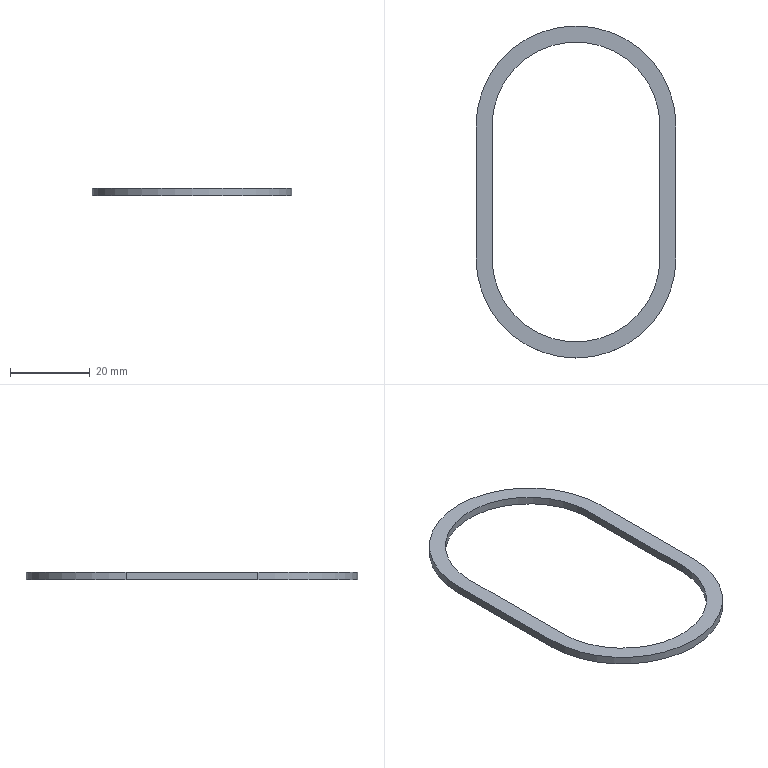Component | NX | 13 | 1 solid | 10 faces | box 50 x 83 x 2 mm | volume 1684 mm3 | plane 6 | cylinder 4 | commonest cylinder face diameters 42 x2 50 x2
STEP:
#1=CARTESIAN_POINT('',(0.,0.,0.));
#2=DIRECTION('',(0.,0.,1.));
#3=DIRECTION('',(1.,0.,0.));
#4=AXIS2_PLACEMENT_3D('',#1,#2,#3);
#5=CARTESIAN_POINT('',(-21.,16.5,30.));
#6=VERTEX_POINT('',#5);
#7=CARTESIAN_POINT('',(-21.,16.5,28.));
#8=VERTEX_POINT('',#7);
#9=CARTESIAN_POINT('',(-21.,16.5,30.));
#10=DIRECTION('',(0.,0.,-1.));
#11=VECTOR('',#10,1.);
#12=LINE('',#9,#11);
#13=CARTESIAN_POINT('',(0.0000016,16.5,30.));
#14=DIRECTION('',(0.,0.,-1.));
#15=DIRECTION('',(0.00000005,1.,0.));
#16=AXIS2_PLACEMENT_3D('',#13,#14,#15);
#17=CYLINDRICAL_SURFACE('',#16,21.);
#18=CARTESIAN_POINT('',(4.712,0.));
#19=DIRECTION('',(0.,1.));
#20=VECTOR('',#19,1.);
#21=LINE('',#18,#20);
#22=(GEOMETRIC_REPRESENTATION_CONTEXT(2)PARAMETRIC_REPRESENTATION_CONTEXT()REPRESENTATION_CONTEXT('',''));
#23=DEFINITIONAL_REPRESENTATION('',(#21),#22);
#24=PCURVE('',#17,#23);
#25=CARTESIAN_POINT('',(-21.,-16.5,30.));
#26=DIRECTION('',(-1.,0.00000005,0.));
#27=DIRECTION('',(-0.00000005,-1.,0.));
#28=AXIS2_PLACEMENT_3D('',#25,#26,#27);
#29=PLANE('',#28);
#30=CARTESIAN_POINT('',(-33.,0.));
#31=DIRECTION('',(0.,-1.));
#32=VECTOR('',#31,1.);
#33=LINE('',#30,#32);
#34=(GEOMETRIC_REPRESENTATION_CONTEXT(2)PARAMETRIC_REPRESENTATION_CONTEXT()REPRESENTATION_CONTEXT('',''));
#35=DEFINITIONAL_REPRESENTATION('',(#33),#34);
#36=PCURVE('',#29,#35);
#37=SURFACE_CURVE('',#12,(#24,#36),.PCURVE_S1.);
#38=EDGE_CURVE('',#6,#8,#37,.T.);
#39=ORIENTED_EDGE('',*,*,#38,.F.);
#40=CARTESIAN_POINT('',(21.,16.5,30.));
#41=VERTEX_POINT('',#40);
#42=CARTESIAN_POINT('',(0.0000016,16.5,30.));
#43=DIRECTION('',(0.,0.,-1.));
#44=DIRECTION('',(-0.00000005,-1.,0.));
#45=AXIS2_PLACEMENT_3D('',#42,#43,#44);
#46=CIRCLE('',#45,21.);
#47=CARTESIAN_POINT('',(3.142,0.));
#48=DIRECTION('',(1.,0.));
#49=VECTOR('',#48,1.);
#50=LINE('',#47,#49);
#51=(GEOMETRIC_REPRESENTATION_CONTEXT(2)PARAMETRIC_REPRESENTATION_CONTEXT()REPRESENTATION_CONTEXT('',''));
#52=DEFINITIONAL_REPRESENTATION('',(#50),#51);
#53=PCURVE('',#17,#52);
#54=CARTESIAN_POINT('',(0.0000016,16.5,30.));
#55=DIRECTION('',(0.,0.,1.));
#56=DIRECTION('',(-0.00000005,-1.,0.));
#57=AXIS2_PLACEMENT_3D('',#54,#55,#56);
#58=PLANE('',#57);
#59=CARTESIAN_POINT('',(21.,0.));
#60=CARTESIAN_POINT('',(21.,-36.373));
#61=CARTESIAN_POINT('',(-10.5,-18.187));
#62=CARTESIAN_POINT('',(-42.,-0.));
#63=CARTESIAN_POINT('',(-10.5,18.187));
#64=CARTESIAN_POINT('',(21.,36.373));
#65=CARTESIAN_POINT('',(21.,0.));
#66=(BOUNDED_CURVE()B_SPLINE_CURVE(2,(#59,#60,#61,#62,#63,#64,#65),.UNSPECIFIED.,.T.,.F.)B_SPLINE_CURVE_WITH_KNOTS((1,2,2,2,2,1),(-2.094,0.,2.094,4.189,6.283,8.378),.UNSPECIFIED.)CURVE()GEOMETRIC_REPRESENTATION_ITEM()RATIONAL_B_SPLINE_CURVE((1.,0.5,1.,0.5,1.,0.5,1.))REPRESENTATION_ITEM(''));
#67=(GEOMETRIC_REPRESENTATION_CONTEXT(2)PARAMETRIC_REPRESENTATION_CONTEXT()REPRESENTATION_CONTEXT('',''));
#68=DEFINITIONAL_REPRESENTATION('',(#66),#67);
#69=PCURVE('',#58,#68);
#70=SURFACE_CURVE('',#46,(#53,#69),.PCURVE_S1.);
#71=EDGE_CURVE('',#6,#41,#70,.T.);
#72=ORIENTED_EDGE('',*,*,#71,.T.);
#73=CARTESIAN_POINT('',(21.,16.5,28.));
#74=VERTEX_POINT('',#73);
#75=CARTESIAN_POINT('',(21.,16.5,30.));
#76=DIRECTION('',(0.,0.,-1.));
#77=VECTOR('',#76,1.);
#78=LINE('',#75,#77);
#79=CARTESIAN_POINT('',(7.854,0.));
#80=DIRECTION('',(0.,1.));
#81=VECTOR('',#80,1.);
#82=LINE('',#79,#81);
#83=(GEOMETRIC_REPRESENTATION_CONTEXT(2)PARAMETRIC_REPRESENTATION_CONTEXT()REPRESENTATION_CONTEXT('',''));
#84=DEFINITIONAL_REPRESENTATION('',(#82),#83);
#85=PCURVE('',#17,#84);
#86=CARTESIAN_POINT('',(21.,16.5,30.));
#87=DIRECTION('',(1.,-0.00000005,0.));
#88=DIRECTION('',(0.00000005,1.,0.));
#89=AXIS2_PLACEMENT_3D('',#86,#87,#88);
#90=PLANE('',#89);
#91=CARTESIAN_POINT('',(0.,0.));
#92=DIRECTION('',(0.,-1.));
#93=VECTOR('',#92,1.);
#94=LINE('',#91,#93);
#95=(GEOMETRIC_REPRESENTATION_CONTEXT(2)PARAMETRIC_REPRESENTATION_CONTEXT()REPRESENTATION_CONTEXT('',''));
#96=DEFINITIONAL_REPRESENTATION('',(#94),#95);
#97=PCURVE('',#90,#96);
#98=SURFACE_CURVE('',#78,(#85,#97),.PCURVE_S1.);
#99=EDGE_CURVE('',#41,#74,#98,.T.);
#100=ORIENTED_EDGE('',*,*,#99,.T.);
#101=CARTESIAN_POINT('',(0.0000016,16.5,28.));
#102=DIRECTION('',(0.,0.,-1.));
#103=DIRECTION('',(-0.00000005,-1.,0.));
#104=AXIS2_PLACEMENT_3D('',#101,#102,#103);
#105=CIRCLE('',#104,21.);
#106=CARTESIAN_POINT('',(3.142,2.));
#107=DIRECTION('',(1.,0.));
#108=VECTOR('',#107,1.);
#109=LINE('',#106,#108);
#110=(GEOMETRIC_REPRESENTATION_CONTEXT(2)PARAMETRIC_REPRESENTATION_CONTEXT()REPRESENTATION_CONTEXT('',''));
#111=DEFINITIONAL_REPRESENTATION('',(#109),#110);
#112=PCURVE('',#17,#111);
#113=CARTESIAN_POINT('',(0.0000016,16.5,28.));
#114=DIRECTION('',(0.,0.,1.));
#115=DIRECTION('',(-0.00000005,-1.,0.));
#116=AXIS2_PLACEMENT_3D('',#113,#114,#115);
#117=PLANE('',#116);
#118=CARTESIAN_POINT('',(21.,0.));
#119=CARTESIAN_POINT('',(21.,-36.373));
#120=CARTESIAN_POINT('',(-10.5,-18.187));
#121=CARTESIAN_POINT('',(-42.,-0.));
#122=CARTESIAN_POINT('',(-10.5,18.187));
#123=CARTESIAN_POINT('',(21.,36.373));
#124=CARTESIAN_POINT('',(21.,0.));
#125=(BOUNDED_CURVE()B_SPLINE_CURVE(2,(#118,#119,#120,#121,#122,#123,#124),.UNSPECIFIED.,.T.,.F.)B_SPLINE_CURVE_WITH_KNOTS((1,2,2,2,2,1),(-2.094,0.,2.094,4.189,6.283,8.378),.UNSPECIFIED.)CURVE()GEOMETRIC_REPRESENTATION_ITEM()RATIONAL_B_SPLINE_CURVE((1.,0.5,1.,0.5,1.,0.5,1.))REPRESENTATION_ITEM(''));
#126=(GEOMETRIC_REPRESENTATION_CONTEXT(2)PARAMETRIC_REPRESENTATION_CONTEXT()REPRESENTATION_CONTEXT('',''));
#127=DEFINITIONAL_REPRESENTATION('',(#125),#126);
#128=PCURVE('',#117,#127);
#129=SURFACE_CURVE('',#105,(#112,#128),.PCURVE_S1.);
#130=EDGE_CURVE('',#8,#74,#129,.T.);
#131=ORIENTED_EDGE('',*,*,#130,.F.);
#132=EDGE_LOOP('',(#39,#72,#100,#131));
#133=FACE_BOUND('',#132,.F.);
#134=ADVANCED_FACE('',(#133),#17,.F.);
#135=CARTESIAN_POINT('',(21.,-16.5,28.));
#136=VERTEX_POINT('',#135);
#137=CARTESIAN_POINT('',(21.,16.5,28.));
#138=DIRECTION('',(-0.00000005,-1.,0.));
#139=VECTOR('',#138,1.);
#140=LINE('',#137,#139);
#141=CARTESIAN_POINT('',(0.,-2.));
#142=DIRECTION('',(-1.,0.));
#143=VECTOR('',#142,1.);
#144=LINE('',#141,#143);
#145=(GEOMETRIC_REPRESENTATION_CONTEXT(2)PARAMETRIC_REPRESENTATION_CONTEXT()REPRESENTATION_CONTEXT('',''));
#146=DEFINITIONAL_REPRESENTATION('',(#144),#145);
#147=PCURVE('',#90,#146);
#148=CARTESIAN_POINT('',(-0.,21.));
#149=DIRECTION('',(1.,-0.));
#150=VECTOR('',#149,1.);
#151=LINE('',#148,#150);
#152=(GEOMETRIC_REPRESENTATION_CONTEXT(2)PARAMETRIC_REPRESENTATION_CONTEXT()REPRESENTATION_CONTEXT('',''));
#153=DEFINITIONAL_REPRESENTATION('',(#151),#152);
#154=PCURVE('',#117,#153);
#155=SURFACE_CURVE('',#140,(#147,#154),.PCURVE_S1.);
#156=EDGE_CURVE('',#74,#136,#155,.T.);
#157=ORIENTED_EDGE('',*,*,#156,.T.);
#158=CARTESIAN_POINT('',(21.,-16.5,30.));
#159=VERTEX_POINT('',#158);
#160=CARTESIAN_POINT('',(21.,-16.5,30.));
#161=DIRECTION('',(0.,0.,-1.));
#162=VECTOR('',#161,1.);
#163=LINE('',#160,#162);
#164=CARTESIAN_POINT('',(-33.,0.));
#165=DIRECTION('',(0.,-1.));
#166=VECTOR('',#165,1.);
#167=LINE('',#164,#166);
#168=(GEOMETRIC_REPRESENTATION_CONTEXT(2)PARAMETRIC_REPRESENTATION_CONTEXT()REPRESENTATION_CONTEXT('',''));
#169=DEFINITIONAL_REPRESENTATION('',(#167),#168);
#170=PCURVE('',#90,#169);
#171=CARTESIAN_POINT('',(-0.,-16.5,30.));
#172=DIRECTION('',(0.,0.,-1.));
#173=DIRECTION('',(0.00000005,1.,0.));
#174=AXIS2_PLACEMENT_3D('',#171,#172,#173);
#175=CYLINDRICAL_SURFACE('',#174,21.);
#176=CARTESIAN_POINT('',(1.571,0.));
#177=DIRECTION('',(0.,1.));
#178=VECTOR('',#177,1.);
#179=LINE('',#176,#178);
#180=(GEOMETRIC_REPRESENTATION_CONTEXT(2)PARAMETRIC_REPRESENTATION_CONTEXT()REPRESENTATION_CONTEXT('',''));
#181=DEFINITIONAL_REPRESENTATION('',(#179),#180);
#182=PCURVE('',#175,#181);
#183=SURFACE_CURVE('',#163,(#170,#182),.PCURVE_S1.);
#184=EDGE_CURVE('',#159,#136,#183,.T.);
#185=ORIENTED_EDGE('',*,*,#184,.F.);
#186=CARTESIAN_POINT('',(21.,16.5,30.));
#187=DIRECTION('',(-0.00000005,-1.,0.));
#188=VECTOR('',#187,1.);
#189=LINE('',#186,#188);
#190=CARTESIAN_POINT('',(0.,0.));
#191=DIRECTION('',(-1.,0.));
#192=VECTOR('',#191,1.);
#193=LINE('',#190,#192);
#194=(GEOMETRIC_REPRESENTATION_CONTEXT(2)PARAMETRIC_REPRESENTATION_CONTEXT()REPRESENTATION_CONTEXT('',''));
#195=DEFINITIONAL_REPRESENTATION('',(#193),#194);
#196=PCURVE('',#90,#195);
#197=CARTESIAN_POINT('',(-0.,21.));
#198=DIRECTION('',(1.,-0.));
#199=VECTOR('',#198,1.);
#200=LINE('',#197,#199);
#201=(GEOMETRIC_REPRESENTATION_CONTEXT(2)PARAMETRIC_REPRESENTATION_CONTEXT()REPRESENTATION_CONTEXT('',''));
#202=DEFINITIONAL_REPRESENTATION('',(#200),#201);
#203=PCURVE('',#58,#202);
#204=SURFACE_CURVE('',#189,(#196,#203),.PCURVE_S1.);
#205=EDGE_CURVE('',#41,#159,#204,.T.);
#206=ORIENTED_EDGE('',*,*,#205,.F.);
#207=ORIENTED_EDGE('',*,*,#99,.T.);
#208=EDGE_LOOP('',(#157,#185,#206,#207));
#209=FACE_BOUND('',#208,.T.);
#210=ADVANCED_FACE('',(#209),#90,.F.);
#211=ORIENTED_EDGE('',*,*,#184,.F.);
#212=CARTESIAN_POINT('',(-21.,-16.5,30.));
#213=VERTEX_POINT('',#212);
#214=CARTESIAN_POINT('',(-0.,-16.5,30.));
#215=DIRECTION('',(0.,0.,-1.));
#216=DIRECTION('',(-0.00000005,-1.,0.));
#217=AXIS2_PLACEMENT_3D('',#214,#215,#216);
#218=CIRCLE('',#217,21.);
#219=CARTESIAN_POINT('',(-3.142,0.));
#220=DIRECTION('',(1.,0.));
#221=VECTOR('',#220,1.);
#222=LINE('',#219,#221);
#223=(GEOMETRIC_REPRESENTATION_CONTEXT(2)PARAMETRIC_REPRESENTATION_CONTEXT()REPRESENTATION_CONTEXT('',''));
#224=DEFINITIONAL_REPRESENTATION('',(#222),#223);
#225=PCURVE('',#175,#224);
#226=CARTESIAN_POINT('',(54.,0.));
#227=CARTESIAN_POINT('',(54.,-36.373));
#228=CARTESIAN_POINT('',(22.5,-18.187));
#229=CARTESIAN_POINT('',(-9.,-0.));
#230=CARTESIAN_POINT('',(22.5,18.187));
#231=CARTESIAN_POINT('',(54.,36.373));
#232=CARTESIAN_POINT('',(54.,0.));
#233=(BOUNDED_CURVE()B_SPLINE_CURVE(2,(#226,#227,#228,#229,#230,#231,#232),.UNSPECIFIED.,.T.,.F.)B_SPLINE_CURVE_WITH_KNOTS((1,2,2,2,2,1),(-2.094,0.,2.094,4.189,6.283,8.378),.UNSPECIFIED.)CURVE()GEOMETRIC_REPRESENTATION_ITEM()RATIONAL_B_SPLINE_CURVE((1.,0.5,1.,0.5,1.,0.5,1.))REPRESENTATION_ITEM(''));
#234=(GEOMETRIC_REPRESENTATION_CONTEXT(2)PARAMETRIC_REPRESENTATION_CONTEXT()REPRESENTATION_CONTEXT('',''));
#235=DEFINITIONAL_REPRESENTATION('',(#233),#234);
#236=PCURVE('',#58,#235);
#237=SURFACE_CURVE('',#218,(#225,#236),.PCURVE_S1.);
#238=EDGE_CURVE('',#159,#213,#237,.T.);
#239=ORIENTED_EDGE('',*,*,#238,.T.);
#240=CARTESIAN_POINT('',(-21.,-16.5,28.));
#241=VERTEX_POINT('',#240);
#242=CARTESIAN_POINT('',(-21.,-16.5,30.));
#243=DIRECTION('',(0.,0.,-1.));
#244=VECTOR('',#243,1.);
#245=LINE('',#242,#244);
#246=CARTESIAN_POINT('',(4.712,0.));
#247=DIRECTION('',(0.,1.));
#248=VECTOR('',#247,1.);
#249=LINE('',#246,#248);
#250=(GEOMETRIC_REPRESENTATION_CONTEXT(2)PARAMETRIC_REPRESENTATION_CONTEXT()REPRESENTATION_CONTEXT('',''));
#251=DEFINITIONAL_REPRESENTATION('',(#249),#250);
#252=PCURVE('',#175,#251);
#253=CARTESIAN_POINT('',(-0.,0.));
#254=DIRECTION('',(0.,-1.));
#255=VECTOR('',#254,1.);
#256=LINE('',#253,#255);
#257=(GEOMETRIC_REPRESENTATION_CONTEXT(2)PARAMETRIC_REPRESENTATION_CONTEXT()REPRESENTATION_CONTEXT('',''));
#258=DEFINITIONAL_REPRESENTATION('',(#256),#257);
#259=PCURVE('',#29,#258);
#260=SURFACE_CURVE('',#245,(#252,#259),.PCURVE_S1.);
#261=EDGE_CURVE('',#213,#241,#260,.T.);
#262=ORIENTED_EDGE('',*,*,#261,.T.);
#263=CARTESIAN_POINT('',(-0.,-16.5,28.));
#264=DIRECTION('',(0.,0.,-1.));
#265=DIRECTION('',(-0.00000005,-1.,0.));
#266=AXIS2_PLACEMENT_3D('',#263,#264,#265);
#267=CIRCLE('',#266,21.);
#268=CARTESIAN_POINT('',(-3.142,2.));
#269=DIRECTION('',(1.,0.));
#270=VECTOR('',#269,1.);
#271=LINE('',#268,#270);
#272=(GEOMETRIC_REPRESENTATION_CONTEXT(2)PARAMETRIC_REPRESENTATION_CONTEXT()REPRESENTATION_CONTEXT('',''));
#273=DEFINITIONAL_REPRESENTATION('',(#271),#272);
#274=PCURVE('',#175,#273);
#275=CARTESIAN_POINT('',(54.,0.));
#276=CARTESIAN_POINT('',(54.,-36.373));
#277=CARTESIAN_POINT('',(22.5,-18.187));
#278=CARTESIAN_POINT('',(-9.,-0.));
#279=CARTESIAN_POINT('',(22.5,18.187));
#280=CARTESIAN_POINT('',(54.,36.373));
#281=CARTESIAN_POINT('',(54.,0.));
#282=(BOUNDED_CURVE()B_SPLINE_CURVE(2,(#275,#276,#277,#278,#279,#280,#281),.UNSPECIFIED.,.T.,.F.)B_SPLINE_CURVE_WITH_KNOTS((1,2,2,2,2,1),(-2.094,0.,2.094,4.189,6.283,8.378),.UNSPECIFIED.)CURVE()GEOMETRIC_REPRESENTATION_ITEM()RATIONAL_B_SPLINE_CURVE((1.,0.5,1.,0.5,1.,0.5,1.))REPRESENTATION_ITEM(''));
#283=(GEOMETRIC_REPRESENTATION_CONTEXT(2)PARAMETRIC_REPRESENTATION_CONTEXT()REPRESENTATION_CONTEXT('',''));
#284=DEFINITIONAL_REPRESENTATION('',(#282),#283);
#285=PCURVE('',#117,#284);
#286=SURFACE_CURVE('',#267,(#274,#285),.PCURVE_S1.);
#287=EDGE_CURVE('',#136,#241,#286,.T.);
#288=ORIENTED_EDGE('',*,*,#287,.F.);
#289=EDGE_LOOP('',(#211,#239,#262,#288));
#290=FACE_BOUND('',#289,.F.);
#291=ADVANCED_FACE('',(#290),#175,.F.);
#292=CARTESIAN_POINT('',(25.,16.5,28.));
#293=VERTEX_POINT('',#292);
#294=CARTESIAN_POINT('',(-25.,16.5,28.));
#295=VERTEX_POINT('',#294);
#296=CARTESIAN_POINT('',(0.0000016,16.5,28.));
#297=DIRECTION('',(0.,0.,1.));
#298=DIRECTION('',(-0.00000005,-1.,0.));
#299=AXIS2_PLACEMENT_3D('',#296,#297,#298);
#300=CIRCLE('',#299,25.);
#301=CARTESIAN_POINT('',(0.0000016,16.5,30.));
#302=DIRECTION('',(0.,0.,-1.));
#303=DIRECTION('',(0.00000005,1.,0.));
#304=AXIS2_PLACEMENT_3D('',#301,#302,#303);
#305=CYLINDRICAL_SURFACE('',#304,25.);
#306=CARTESIAN_POINT('',(3.142,2.));
#307=DIRECTION('',(-1.,0.));
#308=VECTOR('',#307,1.);
#309=LINE('',#306,#308);
#310=(GEOMETRIC_REPRESENTATION_CONTEXT(2)PARAMETRIC_REPRESENTATION_CONTEXT()REPRESENTATION_CONTEXT('',''));
#311=DEFINITIONAL_REPRESENTATION('',(#309),#310);
#312=PCURVE('',#305,#311);
#313=CARTESIAN_POINT('',(0.,0.));
#314=DIRECTION('',(1.,0.));
#315=AXIS2_PLACEMENT_2D('',#313,#314);
#316=CIRCLE('',#315,25.);
#317=(GEOMETRIC_REPRESENTATION_CONTEXT(2)PARAMETRIC_REPRESENTATION_CONTEXT()REPRESENTATION_CONTEXT('',''));
#318=DEFINITIONAL_REPRESENTATION('',(#316),#317);
#319=PCURVE('',#117,#318);
#320=SURFACE_CURVE('',#300,(#312,#319),.PCURVE_S1.);
#321=EDGE_CURVE('',#293,#295,#320,.T.);
#322=ORIENTED_EDGE('',*,*,#321,.T.);
#323=CARTESIAN_POINT('',(-25.,16.5,30.));
#324=VERTEX_POINT('',#323);
#325=CARTESIAN_POINT('',(-25.,16.5,30.));
#326=DIRECTION('',(0.,0.,-1.));
#327=VECTOR('',#326,1.);
#328=LINE('',#325,#327);
#329=CARTESIAN_POINT('',(-1.571,0.));
#330=DIRECTION('',(0.,1.));
#331=VECTOR('',#330,1.);
#332=LINE('',#329,#331);
#333=(GEOMETRIC_REPRESENTATION_CONTEXT(2)PARAMETRIC_REPRESENTATION_CONTEXT()REPRESENTATION_CONTEXT('',''));
#334=DEFINITIONAL_REPRESENTATION('',(#332),#333);
#335=PCURVE('',#305,#334);
#336=CARTESIAN_POINT('',(-25.,16.5,30.));
#337=DIRECTION('',(1.,-0.00000005,0.));
#338=DIRECTION('',(0.00000005,1.,0.));
#339=AXIS2_PLACEMENT_3D('',#336,#337,#338);
#340=PLANE('',#339);
#341=CARTESIAN_POINT('',(-0.,0.));
#342=DIRECTION('',(0.,-1.));
#343=VECTOR('',#342,1.);
#344=LINE('',#341,#343);
#345=(GEOMETRIC_REPRESENTATION_CONTEXT(2)PARAMETRIC_REPRESENTATION_CONTEXT()REPRESENTATION_CONTEXT('',''));
#346=DEFINITIONAL_REPRESENTATION('',(#344),#345);
#347=PCURVE('',#340,#346);
#348=SURFACE_CURVE('',#328,(#335,#347),.PCURVE_S1.);
#349=EDGE_CURVE('',#324,#295,#348,.T.);
#350=ORIENTED_EDGE('',*,*,#349,.F.);
#351=CARTESIAN_POINT('',(25.,16.5,30.));
#352=VERTEX_POINT('',#351);
#353=CARTESIAN_POINT('',(0.0000016,16.5,30.));
#354=DIRECTION('',(0.,0.,1.));
#355=DIRECTION('',(-0.00000005,-1.,0.));
#356=AXIS2_PLACEMENT_3D('',#353,#354,#355);
#357=CIRCLE('',#356,25.);
#358=CARTESIAN_POINT('',(3.142,0.));
#359=DIRECTION('',(-1.,0.));
#360=VECTOR('',#359,1.);
#361=LINE('',#358,#360);
#362=(GEOMETRIC_REPRESENTATION_CONTEXT(2)PARAMETRIC_REPRESENTATION_CONTEXT()REPRESENTATION_CONTEXT('',''));
#363=DEFINITIONAL_REPRESENTATION('',(#361),#362);
#364=PCURVE('',#305,#363);
#365=CARTESIAN_POINT('',(0.,0.));
#366=DIRECTION('',(1.,0.));
#367=AXIS2_PLACEMENT_2D('',#365,#366);
#368=CIRCLE('',#367,25.);
#369=(GEOMETRIC_REPRESENTATION_CONTEXT(2)PARAMETRIC_REPRESENTATION_CONTEXT()REPRESENTATION_CONTEXT('',''));
#370=DEFINITIONAL_REPRESENTATION('',(#368),#369);
#371=PCURVE('',#58,#370);
#372=SURFACE_CURVE('',#357,(#364,#371),.PCURVE_S1.);
#373=EDGE_CURVE('',#352,#324,#372,.T.);
#374=ORIENTED_EDGE('',*,*,#373,.F.);
#375=CARTESIAN_POINT('',(25.,16.5,30.));
#376=DIRECTION('',(0.,0.,-1.));
#377=VECTOR('',#376,1.);
#378=LINE('',#375,#377);
#379=CARTESIAN_POINT('',(1.571,0.));
#380=DIRECTION('',(0.,1.));
#381=VECTOR('',#380,1.);
#382=LINE('',#379,#381);
#383=(GEOMETRIC_REPRESENTATION_CONTEXT(2)PARAMETRIC_REPRESENTATION_CONTEXT()REPRESENTATION_CONTEXT('',''));
#384=DEFINITIONAL_REPRESENTATION('',(#382),#383);
#385=PCURVE('',#305,#384);
#386=CARTESIAN_POINT('',(25.,-16.5,30.));
#387=DIRECTION('',(-1.,0.00000005,0.));
#388=DIRECTION('',(-0.00000005,-1.,0.));
#389=AXIS2_PLACEMENT_3D('',#386,#387,#388);
#390=PLANE('',#389);
#391=CARTESIAN_POINT('',(-33.,0.));
#392=DIRECTION('',(0.,-1.));
#393=VECTOR('',#392,1.);
#394=LINE('',#391,#393);
#395=(GEOMETRIC_REPRESENTATION_CONTEXT(2)PARAMETRIC_REPRESENTATION_CONTEXT()REPRESENTATION_CONTEXT('',''));
#396=DEFINITIONAL_REPRESENTATION('',(#394),#395);
#397=PCURVE('',#390,#396);
#398=SURFACE_CURVE('',#378,(#385,#397),.PCURVE_S1.);
#399=EDGE_CURVE('',#352,#293,#398,.T.);
#400=ORIENTED_EDGE('',*,*,#399,.T.);
#401=EDGE_LOOP('',(#322,#350,#374,#400));
#402=FACE_BOUND('',#401,.T.);
#403=ADVANCED_FACE('',(#402),#305,.T.);
#404=CARTESIAN_POINT('',(-25.,-16.5,28.));
#405=VERTEX_POINT('',#404);
#406=CARTESIAN_POINT('',(-25.,16.5,28.));
#407=DIRECTION('',(-0.00000005,-1.,0.));
#408=VECTOR('',#407,1.);
#409=LINE('',#406,#408);
#410=CARTESIAN_POINT('',(0.,-2.));
#411=DIRECTION('',(-1.,0.));
#412=VECTOR('',#411,1.);
#413=LINE('',#410,#412);
#414=(GEOMETRIC_REPRESENTATION_CONTEXT(2)PARAMETRIC_REPRESENTATION_CONTEXT()REPRESENTATION_CONTEXT('',''));
#415=DEFINITIONAL_REPRESENTATION('',(#413),#414);
#416=PCURVE('',#340,#415);
#417=CARTESIAN_POINT('',(-0.,-25.));
#418=DIRECTION('',(1.,0.));
#419=VECTOR('',#418,1.);
#420=LINE('',#417,#419);
#421=(GEOMETRIC_REPRESENTATION_CONTEXT(2)PARAMETRIC_REPRESENTATION_CONTEXT()REPRESENTATION_CONTEXT('',''));
#422=DEFINITIONAL_REPRESENTATION('',(#420),#421);
#423=PCURVE('',#117,#422);
#424=SURFACE_CURVE('',#409,(#416,#423),.PCURVE_S1.);
#425=EDGE_CURVE('',#295,#405,#424,.T.);
#426=ORIENTED_EDGE('',*,*,#425,.T.);
#427=CARTESIAN_POINT('',(-25.,-16.5,30.));
#428=VERTEX_POINT('',#427);
#429=CARTESIAN_POINT('',(-25.,-16.5,30.));
#430=DIRECTION('',(0.,0.,-1.));
#431=VECTOR('',#430,1.);
#432=LINE('',#429,#431);
#433=CARTESIAN_POINT('',(-33.,0.));
#434=DIRECTION('',(0.,-1.));
#435=VECTOR('',#434,1.);
#436=LINE('',#433,#435);
#437=(GEOMETRIC_REPRESENTATION_CONTEXT(2)PARAMETRIC_REPRESENTATION_CONTEXT()REPRESENTATION_CONTEXT('',''));
#438=DEFINITIONAL_REPRESENTATION('',(#436),#437);
#439=PCURVE('',#340,#438);
#440=CARTESIAN_POINT('',(-0.,-16.5,30.));
#441=DIRECTION('',(0.,0.,-1.));
#442=DIRECTION('',(0.00000005,1.,0.));
#443=AXIS2_PLACEMENT_3D('',#440,#441,#442);
#444=CYLINDRICAL_SURFACE('',#443,25.);
#445=CARTESIAN_POINT('',(4.712,0.));
#446=DIRECTION('',(0.,1.));
#447=VECTOR('',#446,1.);
#448=LINE('',#445,#447);
#449=(GEOMETRIC_REPRESENTATION_CONTEXT(2)PARAMETRIC_REPRESENTATION_CONTEXT()REPRESENTATION_CONTEXT('',''));
#450=DEFINITIONAL_REPRESENTATION('',(#448),#449);
#451=PCURVE('',#444,#450);
#452=SURFACE_CURVE('',#432,(#439,#451),.PCURVE_S1.);
#453=EDGE_CURVE('',#428,#405,#452,.T.);
#454=ORIENTED_EDGE('',*,*,#453,.F.);
#455=CARTESIAN_POINT('',(-25.,16.5,30.));
#456=DIRECTION('',(-0.00000005,-1.,0.));
#457=VECTOR('',#456,1.);
#458=LINE('',#455,#457);
#459=CARTESIAN_POINT('',(0.,0.));
#460=DIRECTION('',(-1.,0.));
#461=VECTOR('',#460,1.);
#462=LINE('',#459,#461);
#463=(GEOMETRIC_REPRESENTATION_CONTEXT(2)PARAMETRIC_REPRESENTATION_CONTEXT()REPRESENTATION_CONTEXT('',''));
#464=DEFINITIONAL_REPRESENTATION('',(#462),#463);
#465=PCURVE('',#340,#464);
#466=CARTESIAN_POINT('',(-0.,-25.));
#467=DIRECTION('',(1.,0.));
#468=VECTOR('',#467,1.);
#469=LINE('',#466,#468);
#470=(GEOMETRIC_REPRESENTATION_CONTEXT(2)PARAMETRIC_REPRESENTATION_CONTEXT()REPRESENTATION_CONTEXT('',''));
#471=DEFINITIONAL_REPRESENTATION('',(#469),#470);
#472=PCURVE('',#58,#471);
#473=SURFACE_CURVE('',#458,(#465,#472),.PCURVE_S1.);
#474=EDGE_CURVE('',#324,#428,#473,.T.);
#475=ORIENTED_EDGE('',*,*,#474,.F.);
#476=ORIENTED_EDGE('',*,*,#349,.T.);
#477=EDGE_LOOP('',(#426,#454,#475,#476));
#478=FACE_BOUND('',#477,.T.);
#479=ADVANCED_FACE('',(#478),#340,.F.);
#480=CARTESIAN_POINT('',(25.,-16.5,28.));
#481=VERTEX_POINT('',#480);
#482=CARTESIAN_POINT('',(-0.,-16.5,28.));
#483=DIRECTION('',(0.,0.,1.));
#484=DIRECTION('',(-0.00000005,-1.,0.));
#485=AXIS2_PLACEMENT_3D('',#482,#483,#484);
#486=CIRCLE('',#485,25.);
#487=CARTESIAN_POINT('',(9.425,2.));
#488=DIRECTION('',(-1.,0.));
#489=VECTOR('',#488,1.);
#490=LINE('',#487,#489);
#491=(GEOMETRIC_REPRESENTATION_CONTEXT(2)PARAMETRIC_REPRESENTATION_CONTEXT()REPRESENTATION_CONTEXT('',''));
#492=DEFINITIONAL_REPRESENTATION('',(#490),#491);
#493=PCURVE('',#444,#492);
#494=CARTESIAN_POINT('',(33.,0.));
#495=DIRECTION('',(1.,0.));
#496=AXIS2_PLACEMENT_2D('',#494,#495);
#497=CIRCLE('',#496,25.);
#498=(GEOMETRIC_REPRESENTATION_CONTEXT(2)PARAMETRIC_REPRESENTATION_CONTEXT()REPRESENTATION_CONTEXT('',''));
#499=DEFINITIONAL_REPRESENTATION('',(#497),#498);
#500=PCURVE('',#117,#499);
#501=SURFACE_CURVE('',#486,(#493,#500),.PCURVE_S1.);
#502=EDGE_CURVE('',#405,#481,#501,.T.);
#503=ORIENTED_EDGE('',*,*,#502,.T.);
#504=CARTESIAN_POINT('',(25.,-16.5,30.));
#505=VERTEX_POINT('',#504);
#506=CARTESIAN_POINT('',(25.,-16.5,30.));
#507=DIRECTION('',(0.,0.,-1.));
#508=VECTOR('',#507,1.);
#509=LINE('',#506,#508);
#510=CARTESIAN_POINT('',(1.571,0.));
#511=DIRECTION('',(0.,1.));
#512=VECTOR('',#511,1.);
#513=LINE('',#510,#512);
#514=(GEOMETRIC_REPRESENTATION_CONTEXT(2)PARAMETRIC_REPRESENTATION_CONTEXT()REPRESENTATION_CONTEXT('',''));
#515=DEFINITIONAL_REPRESENTATION('',(#513),#514);
#516=PCURVE('',#444,#515);
#517=CARTESIAN_POINT('',(-0.,0.));
#518=DIRECTION('',(0.,-1.));
#519=VECTOR('',#518,1.);
#520=LINE('',#517,#519);
#521=(GEOMETRIC_REPRESENTATION_CONTEXT(2)PARAMETRIC_REPRESENTATION_CONTEXT()REPRESENTATION_CONTEXT('',''));
#522=DEFINITIONAL_REPRESENTATION('',(#520),#521);
#523=PCURVE('',#390,#522);
#524=SURFACE_CURVE('',#509,(#516,#523),.PCURVE_S1.);
#525=EDGE_CURVE('',#505,#481,#524,.T.);
#526=ORIENTED_EDGE('',*,*,#525,.F.);
#527=CARTESIAN_POINT('',(-0.,-16.5,30.));
#528=DIRECTION('',(0.,0.,1.));
#529=DIRECTION('',(-0.00000005,-1.,0.));
#530=AXIS2_PLACEMENT_3D('',#527,#528,#529);
#531=CIRCLE('',#530,25.);
#532=CARTESIAN_POINT('',(9.425,0.));
#533=DIRECTION('',(-1.,0.));
#534=VECTOR('',#533,1.);
#535=LINE('',#532,#534);
#536=(GEOMETRIC_REPRESENTATION_CONTEXT(2)PARAMETRIC_REPRESENTATION_CONTEXT()REPRESENTATION_CONTEXT('',''));
#537=DEFINITIONAL_REPRESENTATION('',(#535),#536);
#538=PCURVE('',#444,#537);
#539=CARTESIAN_POINT('',(33.,0.));
#540=DIRECTION('',(1.,0.));
#541=AXIS2_PLACEMENT_2D('',#539,#540);
#542=CIRCLE('',#541,25.);
#543=(GEOMETRIC_REPRESENTATION_CONTEXT(2)PARAMETRIC_REPRESENTATION_CONTEXT()REPRESENTATION_CONTEXT('',''));
#544=DEFINITIONAL_REPRESENTATION('',(#542),#543);
#545=PCURVE('',#58,#544);
#546=SURFACE_CURVE('',#531,(#538,#545),.PCURVE_S1.);
#547=EDGE_CURVE('',#428,#505,#546,.T.);
#548=ORIENTED_EDGE('',*,*,#547,.F.);
#549=ORIENTED_EDGE('',*,*,#453,.T.);
#550=EDGE_LOOP('',(#503,#526,#548,#549));
#551=FACE_BOUND('',#550,.T.);
#552=ADVANCED_FACE('',(#551),#444,.T.);
#553=CARTESIAN_POINT('',(25.,-16.5,28.));
#554=DIRECTION('',(0.00000005,1.,0.));
#555=VECTOR('',#554,1.);
#556=LINE('',#553,#555);
#557=CARTESIAN_POINT('',(0.,-2.));
#558=DIRECTION('',(-1.,0.));
#559=VECTOR('',#558,1.);
#560=LINE('',#557,#559);
#561=(GEOMETRIC_REPRESENTATION_CONTEXT(2)PARAMETRIC_REPRESENTATION_CONTEXT()REPRESENTATION_CONTEXT('',''));
#562=DEFINITIONAL_REPRESENTATION('',(#560),#561);
#563=PCURVE('',#390,#562);
#564=CARTESIAN_POINT('',(33.,25.));
#565=DIRECTION('',(-1.,0.));
#566=VECTOR('',#565,1.);
#567=LINE('',#564,#566);
#568=(GEOMETRIC_REPRESENTATION_CONTEXT(2)PARAMETRIC_REPRESENTATION_CONTEXT()REPRESENTATION_CONTEXT('',''));
#569=DEFINITIONAL_REPRESENTATION('',(#567),#568);
#570=PCURVE('',#117,#569);
#571=SURFACE_CURVE('',#556,(#563,#570),.PCURVE_S1.);
#572=EDGE_CURVE('',#481,#293,#571,.T.);
#573=ORIENTED_EDGE('',*,*,#572,.T.);
#574=ORIENTED_EDGE('',*,*,#399,.F.);
#575=CARTESIAN_POINT('',(25.,-16.5,30.));
#576=DIRECTION('',(0.00000005,1.,0.));
#577=VECTOR('',#576,1.);
#578=LINE('',#575,#577);
#579=CARTESIAN_POINT('',(0.,0.));
#580=DIRECTION('',(-1.,0.));
#581=VECTOR('',#580,1.);
#582=LINE('',#579,#581);
#583=(GEOMETRIC_REPRESENTATION_CONTEXT(2)PARAMETRIC_REPRESENTATION_CONTEXT()REPRESENTATION_CONTEXT('',''));
#584=DEFINITIONAL_REPRESENTATION('',(#582),#583);
#585=PCURVE('',#390,#584);
#586=CARTESIAN_POINT('',(33.,25.));
#587=DIRECTION('',(-1.,0.));
#588=VECTOR('',#587,1.);
#589=LINE('',#586,#588);
#590=(GEOMETRIC_REPRESENTATION_CONTEXT(2)PARAMETRIC_REPRESENTATION_CONTEXT()REPRESENTATION_CONTEXT('',''));
#591=DEFINITIONAL_REPRESENTATION('',(#589),#590);
#592=PCURVE('',#58,#591);
#593=SURFACE_CURVE('',#578,(#585,#592),.PCURVE_S1.);
#594=EDGE_CURVE('',#505,#352,#593,.T.);
#595=ORIENTED_EDGE('',*,*,#594,.F.);
#596=ORIENTED_EDGE('',*,*,#525,.T.);
#597=EDGE_LOOP('',(#573,#574,#595,#596));
#598=FACE_BOUND('',#597,.T.);
#599=ADVANCED_FACE('',(#598),#390,.F.);
#600=CARTESIAN_POINT('',(-21.,-16.5,28.));
#601=DIRECTION('',(0.00000005,1.,0.));
#602=VECTOR('',#601,1.);
#603=LINE('',#600,#602);
#604=CARTESIAN_POINT('',(0.,-2.));
#605=DIRECTION('',(-1.,0.));
#606=VECTOR('',#605,1.);
#607=LINE('',#604,#606);
#608=(GEOMETRIC_REPRESENTATION_CONTEXT(2)PARAMETRIC_REPRESENTATION_CONTEXT()REPRESENTATION_CONTEXT('',''));
#609=DEFINITIONAL_REPRESENTATION('',(#607),#608);
#610=PCURVE('',#29,#609);
#611=CARTESIAN_POINT('',(33.,-21.));
#612=DIRECTION('',(-1.,-0.));
#613=VECTOR('',#612,1.);
#614=LINE('',#611,#613);
#615=(GEOMETRIC_REPRESENTATION_CONTEXT(2)PARAMETRIC_REPRESENTATION_CONTEXT()REPRESENTATION_CONTEXT('',''));
#616=DEFINITIONAL_REPRESENTATION('',(#614),#615);
#617=PCURVE('',#117,#616);
#618=SURFACE_CURVE('',#603,(#610,#617),.PCURVE_S1.);
#619=EDGE_CURVE('',#241,#8,#618,.T.);
#620=ORIENTED_EDGE('',*,*,#619,.T.);
#621=ORIENTED_EDGE('',*,*,#38,.F.);
#622=CARTESIAN_POINT('',(-21.,-16.5,30.));
#623=DIRECTION('',(0.00000005,1.,0.));
#624=VECTOR('',#623,1.);
#625=LINE('',#622,#624);
#626=CARTESIAN_POINT('',(0.,0.));
#627=DIRECTION('',(-1.,0.));
#628=VECTOR('',#627,1.);
#629=LINE('',#626,#628);
#630=(GEOMETRIC_REPRESENTATION_CONTEXT(2)PARAMETRIC_REPRESENTATION_CONTEXT()REPRESENTATION_CONTEXT('',''));
#631=DEFINITIONAL_REPRESENTATION('',(#629),#630);
#632=PCURVE('',#29,#631);
#633=CARTESIAN_POINT('',(33.,-21.));
#634=DIRECTION('',(-1.,-0.));
#635=VECTOR('',#634,1.);
#636=LINE('',#633,#635);
#637=(GEOMETRIC_REPRESENTATION_CONTEXT(2)PARAMETRIC_REPRESENTATION_CONTEXT()REPRESENTATION_CONTEXT('',''));
#638=DEFINITIONAL_REPRESENTATION('',(#636),#637);
#639=PCURVE('',#58,#638);
#640=SURFACE_CURVE('',#625,(#632,#639),.PCURVE_S1.);
#641=EDGE_CURVE('',#213,#6,#640,.T.);
#642=ORIENTED_EDGE('',*,*,#641,.F.);
#643=ORIENTED_EDGE('',*,*,#261,.T.);
#644=EDGE_LOOP('',(#620,#621,#642,#643));
#645=FACE_BOUND('',#644,.T.);
#646=ADVANCED_FACE('',(#645),#29,.F.);
#647=ORIENTED_EDGE('',*,*,#373,.T.);
#648=ORIENTED_EDGE('',*,*,#474,.T.);
#649=ORIENTED_EDGE('',*,*,#547,.T.);
#650=ORIENTED_EDGE('',*,*,#594,.T.);
#651=EDGE_LOOP('',(#647,#648,#649,#650));
#652=FACE_BOUND('',#651,.T.);
#653=ORIENTED_EDGE('',*,*,#71,.T.);
#654=ORIENTED_EDGE('',*,*,#205,.T.);
#655=ORIENTED_EDGE('',*,*,#238,.T.);
#656=ORIENTED_EDGE('',*,*,#641,.T.);
#657=EDGE_LOOP('',(#653,#654,#655,#656));
#658=FACE_BOUND('',#657,.T.);
#659=ADVANCED_FACE('',(#652,#658),#58,.T.);
#660=ORIENTED_EDGE('',*,*,#321,.F.);
#661=ORIENTED_EDGE('',*,*,#572,.F.);
#662=ORIENTED_EDGE('',*,*,#502,.F.);
#663=ORIENTED_EDGE('',*,*,#425,.F.);
#664=EDGE_LOOP('',(#660,#661,#662,#663));
#665=FACE_BOUND('',#664,.T.);
#666=ORIENTED_EDGE('',*,*,#130,.F.);
#667=ORIENTED_EDGE('',*,*,#619,.F.);
#668=ORIENTED_EDGE('',*,*,#287,.F.);
#669=ORIENTED_EDGE('',*,*,#156,.F.);
#670=EDGE_LOOP('',(#666,#667,#668,#669));
#671=FACE_BOUND('',#670,.T.);
#672=ADVANCED_FACE('',(#665,#671),#117,.F.);
#673=CLOSED_SHELL('',(#134,#210,#291,#403,#479,#552,#599,#646,#659,#672));
#674=MANIFOLD_SOLID_BREP('',#673);
#675=(LENGTH_UNIT()NAMED_UNIT(*)SI_UNIT(.MILLI.,.METRE.));
#676=UNCERTAINTY_MEASURE_WITH_UNIT(LENGTH_MEASURE(0.0000001),#675,'','');
#677=(NAMED_UNIT(*)PLANE_ANGLE_UNIT()SI_UNIT($,.RADIAN.));
#678=(NAMED_UNIT(*)SI_UNIT($,.STERADIAN.)SOLID_ANGLE_UNIT());
#679=(GEOMETRIC_REPRESENTATION_CONTEXT(3)GLOBAL_UNCERTAINTY_ASSIGNED_CONTEXT((#676))GLOBAL_UNIT_ASSIGNED_CONTEXT((#675,#677,#678))REPRESENTATION_CONTEXT('',''));
#680=ADVANCED_BREP_SHAPE_REPRESENTATION('',(#4,#674),#679);